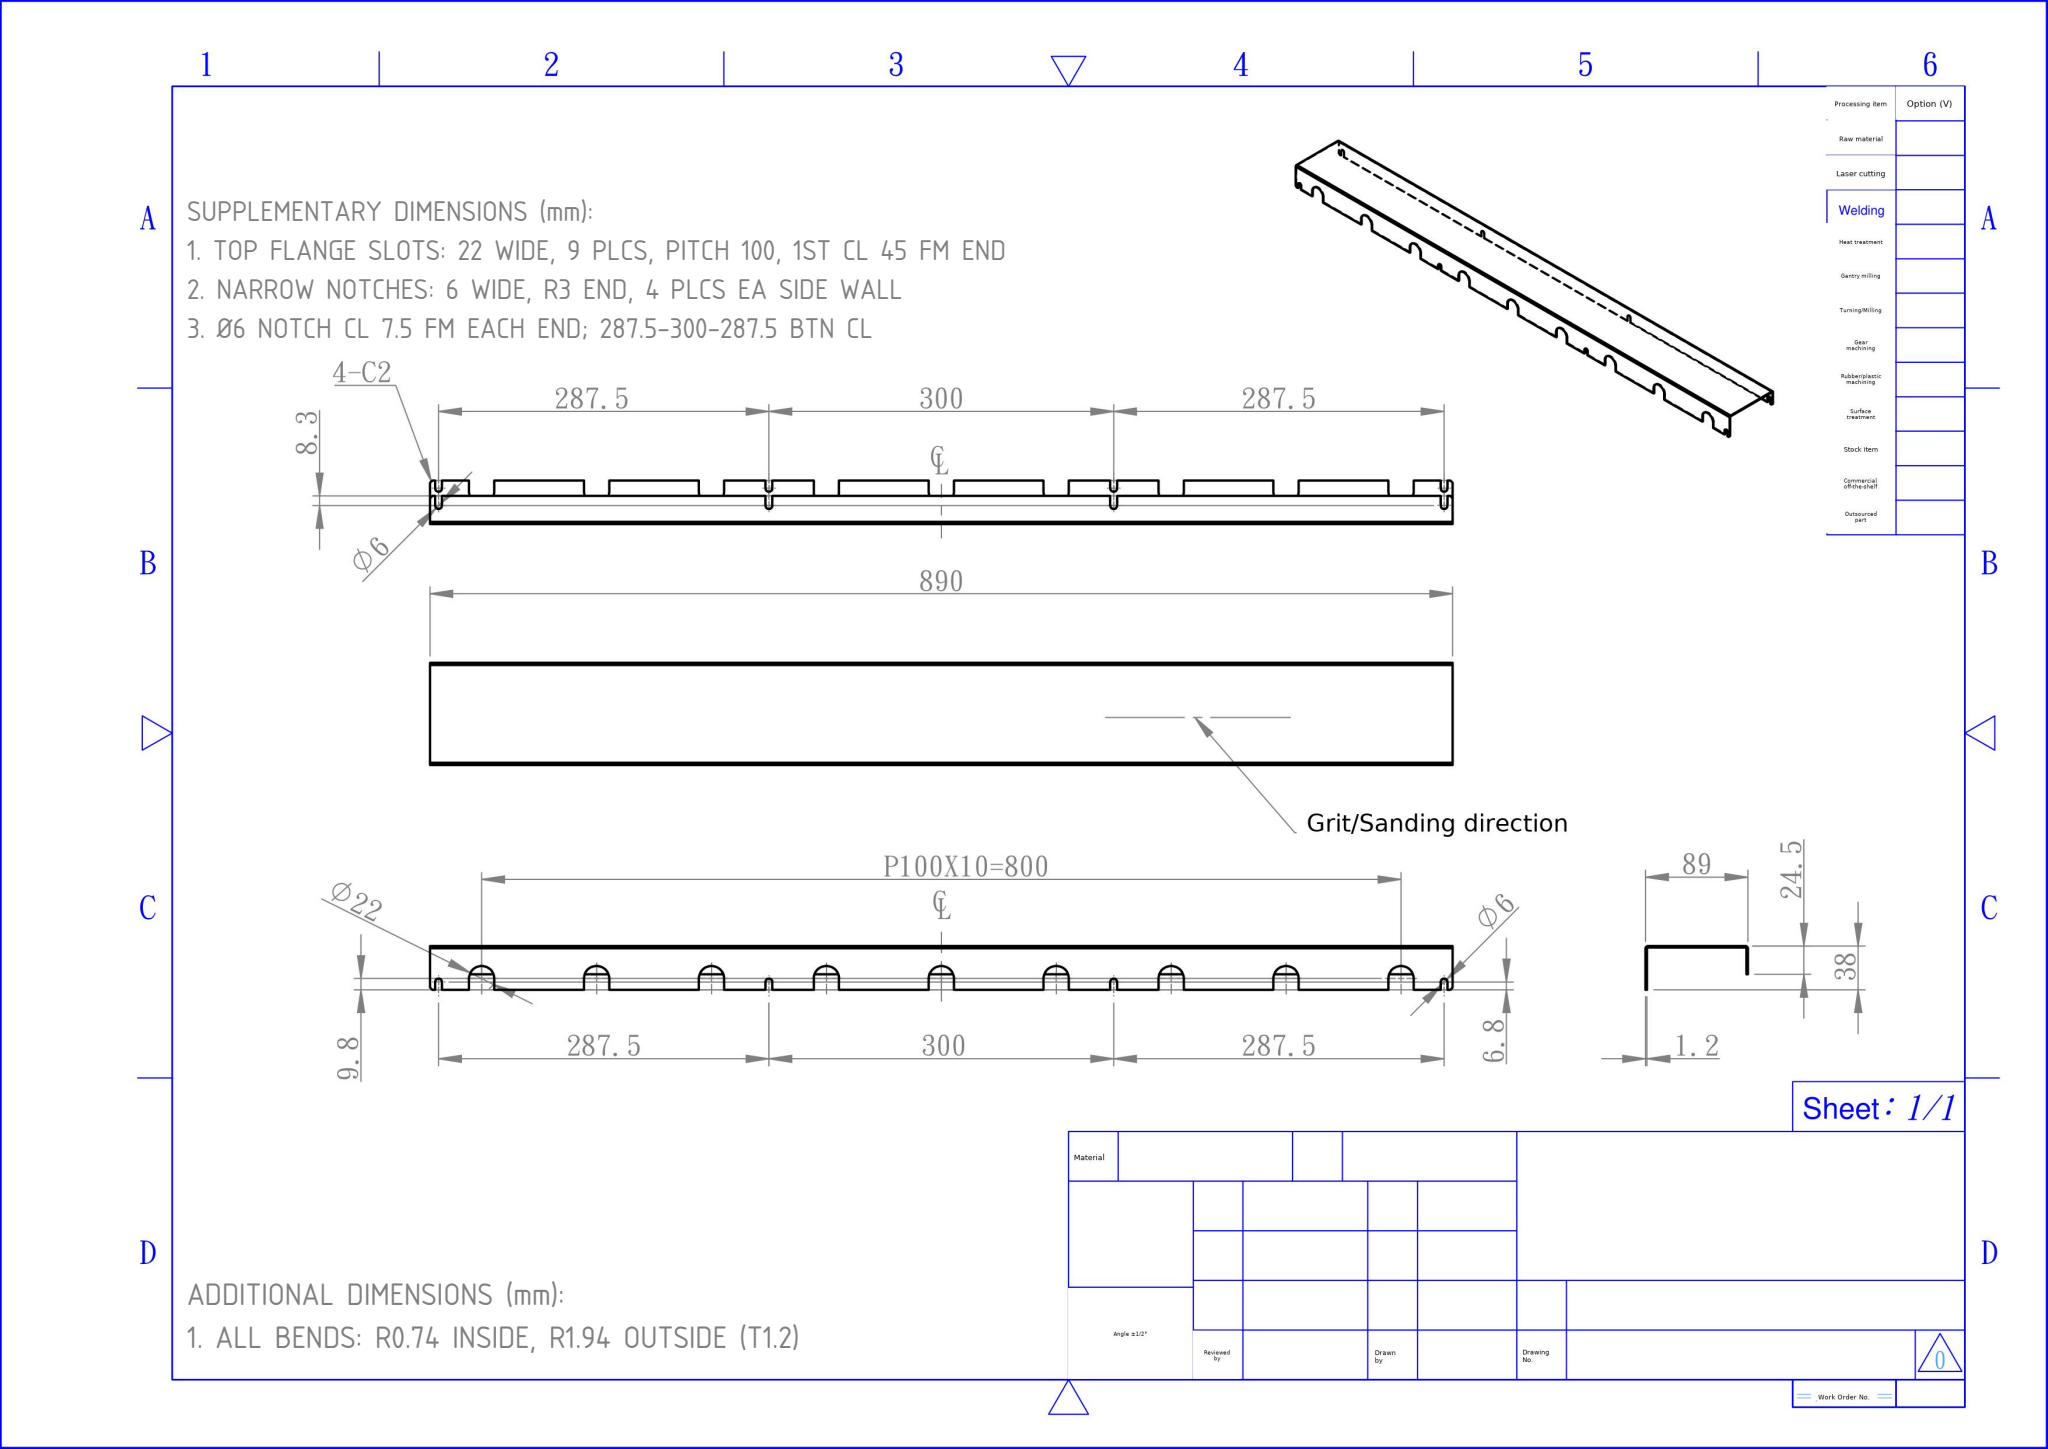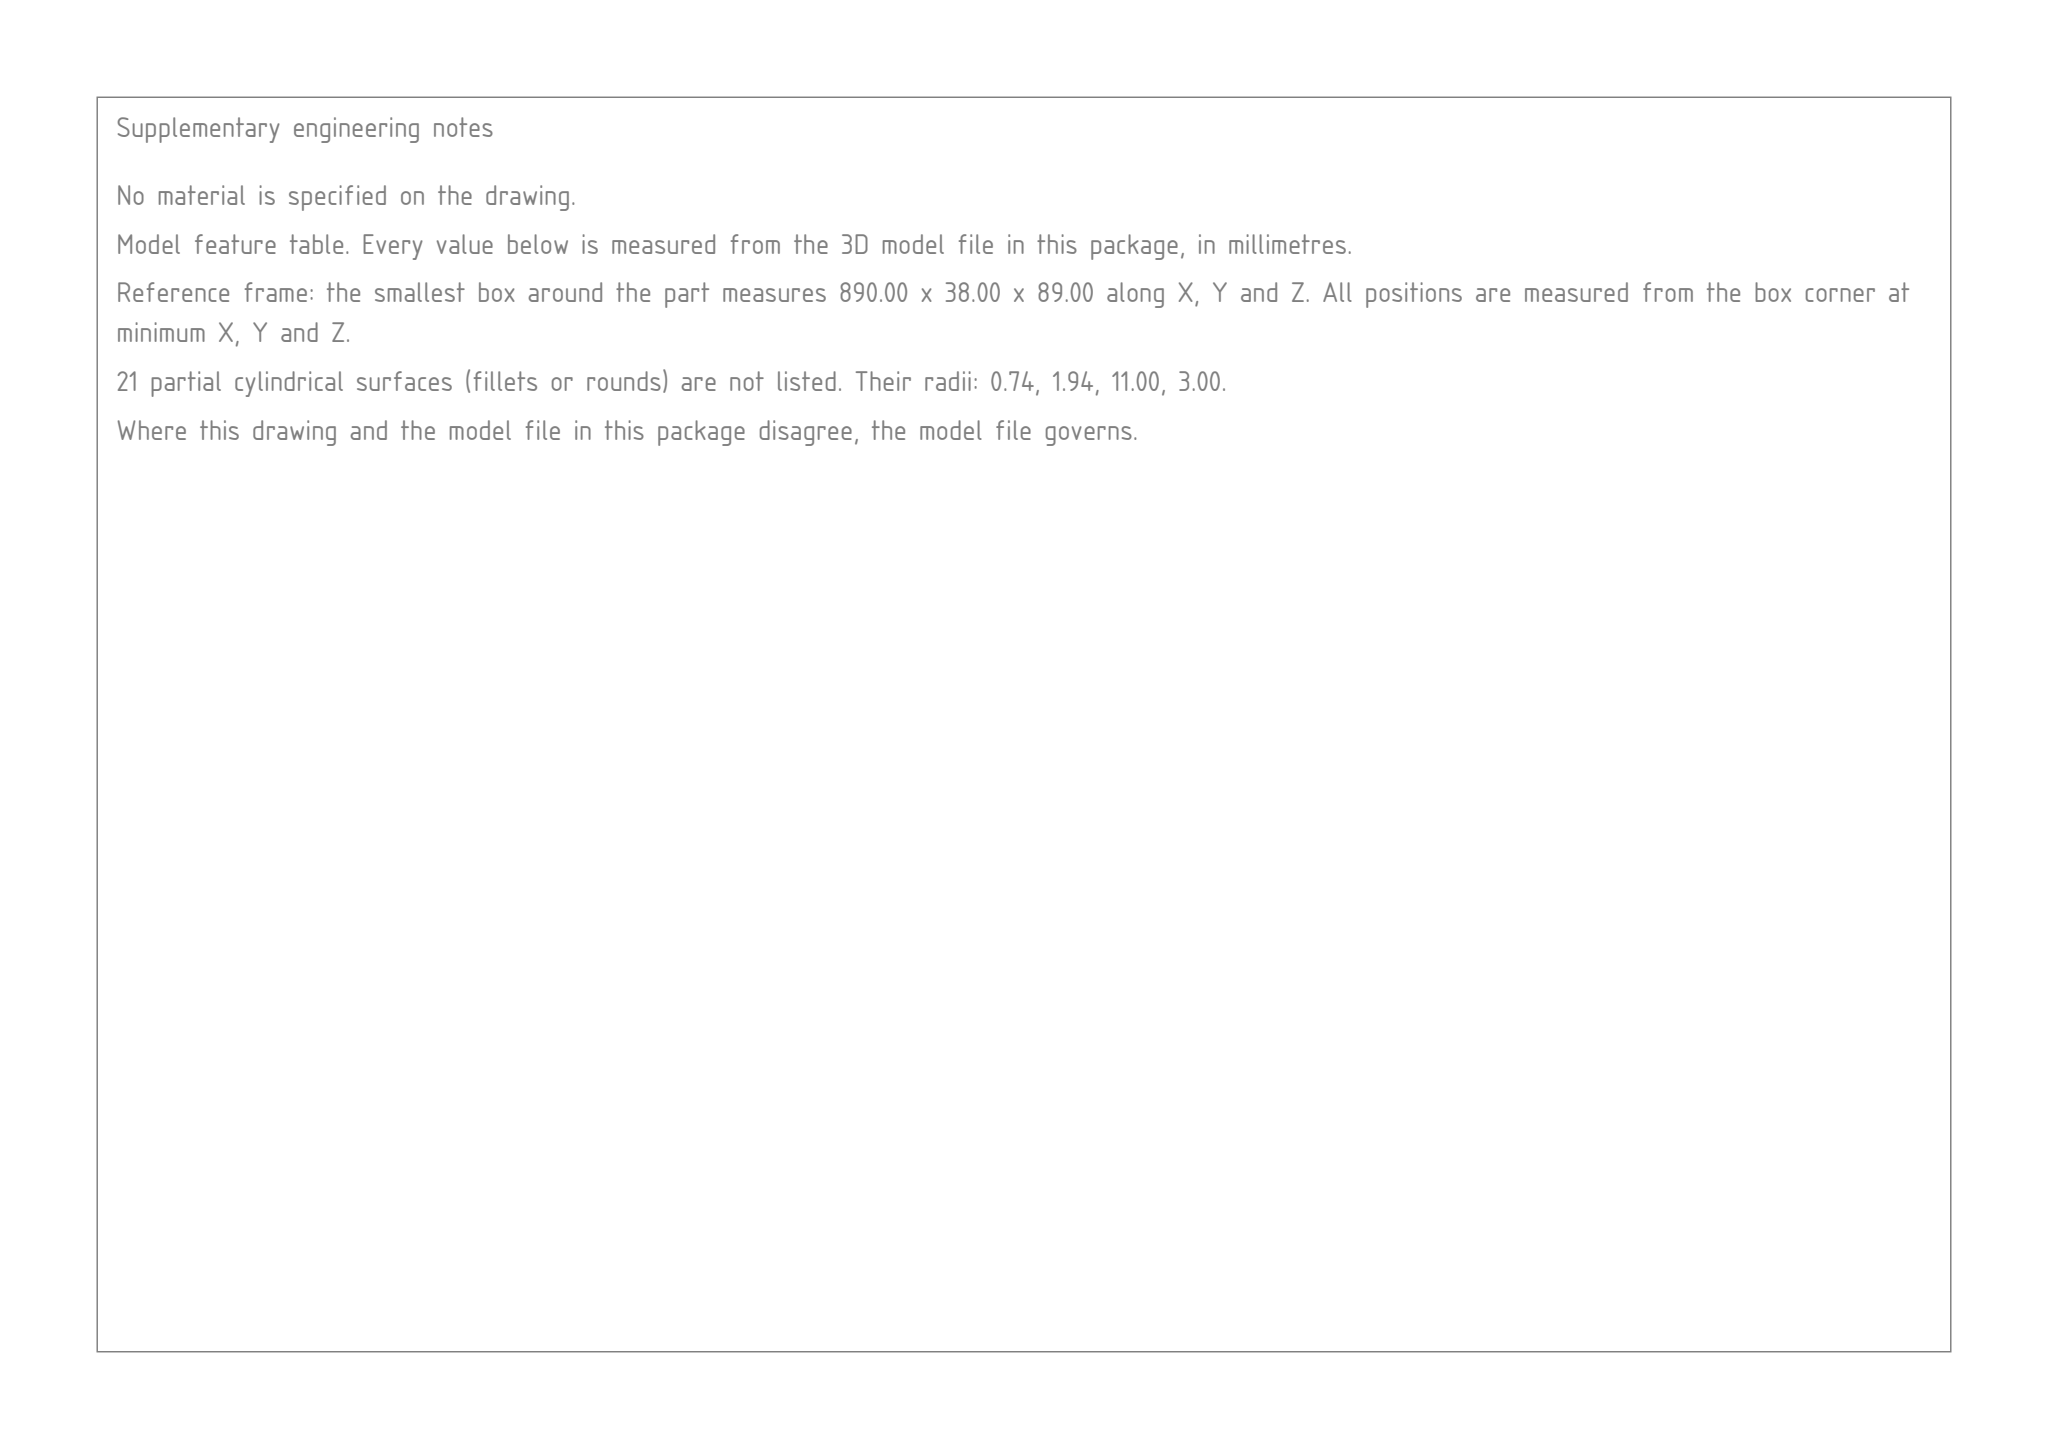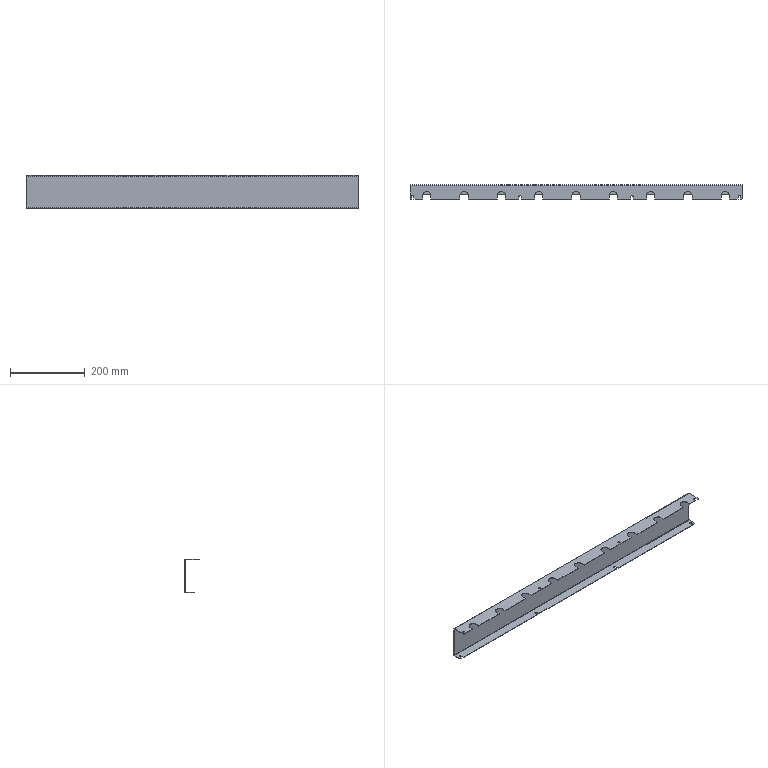Part | SolidWorks | mm | 1 solid | 98 faces | box 890 x 38 x 89 mm | volume 153052 mm3 | plane 73 | cylinder 25 | commonest cylinder face diameters 6 x12 22 x9 3.873 x2 1.473 x2